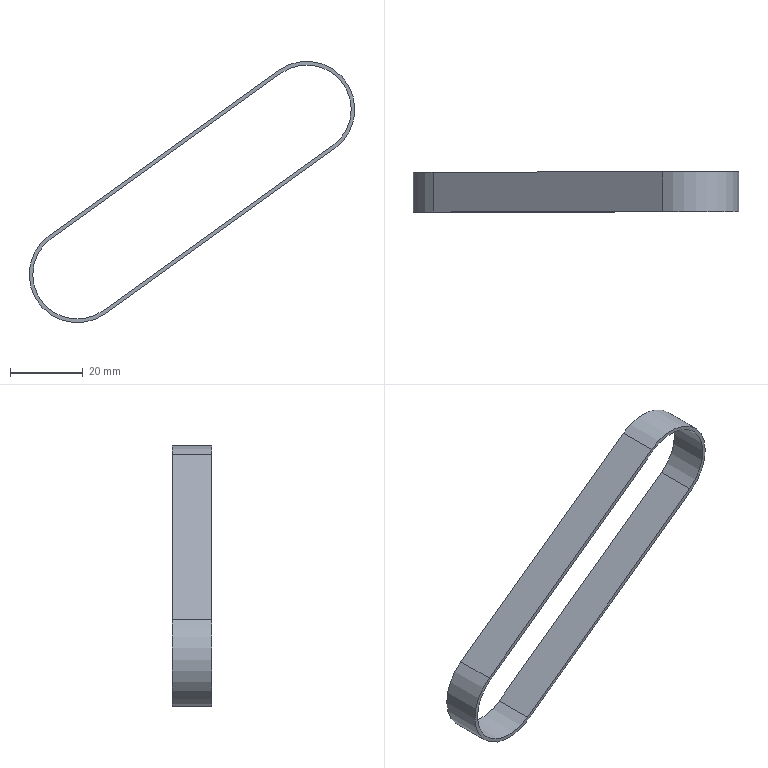Component | NX | BELT | 1 solid | 10 faces | box 89.82 x 11 x 72.05 mm | volume 2597 mm3 | plane 6 | cylinder 4 | commonest cylinder face diameters 26.5 x2 24.5 x2
STEP:
#1=CARTESIAN_POINT('',(0.,0.,0.));
#2=DIRECTION('',(0.,0.,1.));
#3=DIRECTION('',(1.,0.,0.));
#4=AXIS2_PLACEMENT_3D('',#1,#2,#3);
#5=CARTESIAN_POINT('',(-439.414,-35.6,389.312));
#6=VERTEX_POINT('',#5);
#7=CARTESIAN_POINT('',(-376.097,-35.6,434.863));
#8=VERTEX_POINT('',#7);
#9=CARTESIAN_POINT('',(-439.414,-35.6,389.312));
#10=DIRECTION('',(0.8118,0.,0.584));
#11=VECTOR('',#10,1.);
#12=LINE('',#9,#11);
#13=CARTESIAN_POINT('',(-438.83,-35.6,388.5));
#14=DIRECTION('',(0.,-1.,0.));
#15=DIRECTION('',(0.8118,0.,0.584));
#16=AXIS2_PLACEMENT_3D('',#13,#14,#15);
#17=PLANE('',#16);
#18=CARTESIAN_POINT('',(-0.,1.));
#19=DIRECTION('',(1.,0.));
#20=VECTOR('',#19,1.);
#21=LINE('',#18,#20);
#22=(GEOMETRIC_REPRESENTATION_CONTEXT(2)PARAMETRIC_REPRESENTATION_CONTEXT()REPRESENTATION_CONTEXT('',''));
#23=DEFINITIONAL_REPRESENTATION('',(#21),#22);
#24=PCURVE('',#17,#23);
#25=CARTESIAN_POINT('',(-439.414,-46.6,389.312));
#26=DIRECTION('',(-0.584,0.,0.8118));
#27=DIRECTION('',(0.,1.,0.));
#28=AXIS2_PLACEMENT_3D('',#25,#26,#27);
#29=PLANE('',#28);
#30=CARTESIAN_POINT('',(11.,0.));
#31=DIRECTION('',(0.,-1.));
#32=VECTOR('',#31,1.);
#33=LINE('',#30,#32);
#34=(GEOMETRIC_REPRESENTATION_CONTEXT(2)PARAMETRIC_REPRESENTATION_CONTEXT()REPRESENTATION_CONTEXT('',''));
#35=DEFINITIONAL_REPRESENTATION('',(#33),#34);
#36=PCURVE('',#29,#35);
#37=SURFACE_CURVE('',#12,(#24,#36),.PCURVE_S1.);
#38=EDGE_CURVE('',#6,#8,#37,.T.);
#39=ORIENTED_EDGE('',*,*,#38,.T.);
#40=CARTESIAN_POINT('',(-360.621,-35.6,413.352));
#41=VERTEX_POINT('',#40);
#42=CARTESIAN_POINT('',(-368.359,-35.6,424.108));
#43=DIRECTION('',(0.,1.,0.));
#44=DIRECTION('',(-0.8118,0.,-0.584));
#45=AXIS2_PLACEMENT_3D('',#42,#43,#44);
#46=CIRCLE('',#45,13.25);
#47=CARTESIAN_POINT('',(64.75,-12.25));
#48=CARTESIAN_POINT('',(64.75,10.7));
#49=CARTESIAN_POINT('',(84.625,-0.7752));
#50=CARTESIAN_POINT('',(104.5,-12.25));
#51=CARTESIAN_POINT('',(84.625,-23.725));
#52=CARTESIAN_POINT('',(64.75,-35.2));
#53=CARTESIAN_POINT('',(64.75,-12.25));
#54=(BOUNDED_CURVE()B_SPLINE_CURVE(2,(#47,#48,#49,#50,#51,#52,#53),.UNSPECIFIED.,.T.,.F.)B_SPLINE_CURVE_WITH_KNOTS((1,2,2,2,2,1),(-2.094,0.,2.094,4.189,6.283,8.378),.UNSPECIFIED.)CURVE()GEOMETRIC_REPRESENTATION_ITEM()RATIONAL_B_SPLINE_CURVE((1.,0.5,1.,0.5,1.,0.5,1.))REPRESENTATION_ITEM(''));
#55=(GEOMETRIC_REPRESENTATION_CONTEXT(2)PARAMETRIC_REPRESENTATION_CONTEXT()REPRESENTATION_CONTEXT('',''));
#56=DEFINITIONAL_REPRESENTATION('',(#54),#55);
#57=PCURVE('',#17,#56);
#58=CARTESIAN_POINT('',(-368.359,-46.6,424.108));
#59=DIRECTION('',(0.,1.,0.));
#60=DIRECTION('',(-0.8118,0.,-0.584));
#61=AXIS2_PLACEMENT_3D('',#58,#59,#60);
#62=CYLINDRICAL_SURFACE('',#61,13.25);
#63=CARTESIAN_POINT('',(0.,11.));
#64=DIRECTION('',(1.,0.));
#65=VECTOR('',#64,1.);
#66=LINE('',#63,#65);
#67=(GEOMETRIC_REPRESENTATION_CONTEXT(2)PARAMETRIC_REPRESENTATION_CONTEXT()REPRESENTATION_CONTEXT('',''));
#68=DEFINITIONAL_REPRESENTATION('',(#66),#67);
#69=PCURVE('',#62,#68);
#70=SURFACE_CURVE('',#46,(#57,#69),.PCURVE_S1.);
#71=EDGE_CURVE('',#8,#41,#70,.T.);
#72=ORIENTED_EDGE('',*,*,#71,.T.);
#73=CARTESIAN_POINT('',(-423.938,-35.6,367.8));
#74=VERTEX_POINT('',#73);
#75=CARTESIAN_POINT('',(-360.621,-35.6,413.352));
#76=DIRECTION('',(-0.8118,0.,-0.584));
#77=VECTOR('',#76,1.);
#78=LINE('',#75,#77);
#79=CARTESIAN_POINT('',(78.,-25.5));
#80=DIRECTION('',(-1.,0.));
#81=VECTOR('',#80,1.);
#82=LINE('',#79,#81);
#83=(GEOMETRIC_REPRESENTATION_CONTEXT(2)PARAMETRIC_REPRESENTATION_CONTEXT()REPRESENTATION_CONTEXT('',''));
#84=DEFINITIONAL_REPRESENTATION('',(#82),#83);
#85=PCURVE('',#17,#84);
#86=CARTESIAN_POINT('',(-360.621,-46.6,413.352));
#87=DIRECTION('',(0.584,0.,-0.8118));
#88=DIRECTION('',(0.,-1.,0.));
#89=AXIS2_PLACEMENT_3D('',#86,#87,#88);
#90=PLANE('',#89);
#91=CARTESIAN_POINT('',(-11.,0.));
#92=DIRECTION('',(0.,1.));
#93=VECTOR('',#92,1.);
#94=LINE('',#91,#93);
#95=(GEOMETRIC_REPRESENTATION_CONTEXT(2)PARAMETRIC_REPRESENTATION_CONTEXT()REPRESENTATION_CONTEXT('',''));
#96=DEFINITIONAL_REPRESENTATION('',(#94),#95);
#97=PCURVE('',#90,#96);
#98=SURFACE_CURVE('',#78,(#85,#97),.PCURVE_S1.);
#99=EDGE_CURVE('',#41,#74,#98,.T.);
#100=ORIENTED_EDGE('',*,*,#99,.T.);
#101=CARTESIAN_POINT('',(-431.676,-35.6,378.556));
#102=DIRECTION('',(0.,1.,0.));
#103=DIRECTION('',(-0.8118,0.,-0.584));
#104=AXIS2_PLACEMENT_3D('',#101,#102,#103);
#105=CIRCLE('',#104,13.25);
#106=CARTESIAN_POINT('',(-13.25,-12.25));
#107=CARTESIAN_POINT('',(-13.25,10.7));
#108=CARTESIAN_POINT('',(6.625,-0.7752));
#109=CARTESIAN_POINT('',(26.5,-12.25));
#110=CARTESIAN_POINT('',(6.625,-23.725));
#111=CARTESIAN_POINT('',(-13.25,-35.2));
#112=CARTESIAN_POINT('',(-13.25,-12.25));
#113=(BOUNDED_CURVE()B_SPLINE_CURVE(2,(#106,#107,#108,#109,#110,#111,#112),.UNSPECIFIED.,.T.,.F.)B_SPLINE_CURVE_WITH_KNOTS((1,2,2,2,2,1),(-2.094,0.,2.094,4.189,6.283,8.378),.UNSPECIFIED.)CURVE()GEOMETRIC_REPRESENTATION_ITEM()RATIONAL_B_SPLINE_CURVE((1.,0.5,1.,0.5,1.,0.5,1.))REPRESENTATION_ITEM(''));
#114=(GEOMETRIC_REPRESENTATION_CONTEXT(2)PARAMETRIC_REPRESENTATION_CONTEXT()REPRESENTATION_CONTEXT('',''));
#115=DEFINITIONAL_REPRESENTATION('',(#113),#114);
#116=PCURVE('',#17,#115);
#117=CARTESIAN_POINT('',(-431.676,-46.6,378.556));
#118=DIRECTION('',(0.,1.,0.));
#119=DIRECTION('',(-0.8118,0.,-0.584));
#120=AXIS2_PLACEMENT_3D('',#117,#118,#119);
#121=CYLINDRICAL_SURFACE('',#120,13.25);
#122=CARTESIAN_POINT('',(0.,11.));
#123=DIRECTION('',(1.,0.));
#124=VECTOR('',#123,1.);
#125=LINE('',#122,#124);
#126=(GEOMETRIC_REPRESENTATION_CONTEXT(2)PARAMETRIC_REPRESENTATION_CONTEXT()REPRESENTATION_CONTEXT('',''));
#127=DEFINITIONAL_REPRESENTATION('',(#125),#126);
#128=PCURVE('',#121,#127);
#129=SURFACE_CURVE('',#105,(#116,#128),.PCURVE_S1.);
#130=EDGE_CURVE('',#74,#6,#129,.T.);
#131=ORIENTED_EDGE('',*,*,#130,.T.);
#132=EDGE_LOOP('',(#39,#72,#100,#131));
#133=FACE_BOUND('',#132,.T.);
#134=CARTESIAN_POINT('',(-438.83,-35.6,388.5));
#135=VERTEX_POINT('',#134);
#136=CARTESIAN_POINT('',(-375.513,-35.6,434.052));
#137=VERTEX_POINT('',#136);
#138=CARTESIAN_POINT('',(-438.83,-35.6,388.5));
#139=DIRECTION('',(0.8118,0.,0.584));
#140=VECTOR('',#139,1.);
#141=LINE('',#138,#140);
#142=CARTESIAN_POINT('',(0.,0.));
#143=DIRECTION('',(1.,0.));
#144=VECTOR('',#143,1.);
#145=LINE('',#142,#144);
#146=(GEOMETRIC_REPRESENTATION_CONTEXT(2)PARAMETRIC_REPRESENTATION_CONTEXT()REPRESENTATION_CONTEXT('',''));
#147=DEFINITIONAL_REPRESENTATION('',(#145),#146);
#148=PCURVE('',#17,#147);
#149=CARTESIAN_POINT('',(-438.83,-46.6,388.5));
#150=DIRECTION('',(-0.584,0.,0.8118));
#151=DIRECTION('',(0.,1.,0.));
#152=AXIS2_PLACEMENT_3D('',#149,#150,#151);
#153=PLANE('',#152);
#154=CARTESIAN_POINT('',(11.,0.));
#155=DIRECTION('',(0.,-1.));
#156=VECTOR('',#155,1.);
#157=LINE('',#154,#156);
#158=(GEOMETRIC_REPRESENTATION_CONTEXT(2)PARAMETRIC_REPRESENTATION_CONTEXT()REPRESENTATION_CONTEXT('',''));
#159=DEFINITIONAL_REPRESENTATION('',(#157),#158);
#160=PCURVE('',#153,#159);
#161=SURFACE_CURVE('',#141,(#148,#160),.PCURVE_S1.);
#162=EDGE_CURVE('',#135,#137,#161,.T.);
#163=ORIENTED_EDGE('',*,*,#162,.F.);
#164=CARTESIAN_POINT('',(-424.522,-35.6,368.612));
#165=VERTEX_POINT('',#164);
#166=CARTESIAN_POINT('',(-431.676,-35.6,378.556));
#167=DIRECTION('',(0.,1.,0.));
#168=DIRECTION('',(-0.8118,0.,-0.584));
#169=AXIS2_PLACEMENT_3D('',#166,#167,#168);
#170=CIRCLE('',#169,12.25);
#171=CARTESIAN_POINT('',(-12.25,-12.25));
#172=CARTESIAN_POINT('',(-12.25,8.968));
#173=CARTESIAN_POINT('',(6.125,-1.641));
#174=CARTESIAN_POINT('',(24.5,-12.25));
#175=CARTESIAN_POINT('',(6.125,-22.859));
#176=CARTESIAN_POINT('',(-12.25,-33.468));
#177=CARTESIAN_POINT('',(-12.25,-12.25));
#178=(BOUNDED_CURVE()B_SPLINE_CURVE(2,(#171,#172,#173,#174,#175,#176,#177),.UNSPECIFIED.,.T.,.F.)B_SPLINE_CURVE_WITH_KNOTS((1,2,2,2,2,1),(-2.094,0.,2.094,4.189,6.283,8.378),.UNSPECIFIED.)CURVE()GEOMETRIC_REPRESENTATION_ITEM()RATIONAL_B_SPLINE_CURVE((1.,0.5,1.,0.5,1.,0.5,1.))REPRESENTATION_ITEM(''));
#179=(GEOMETRIC_REPRESENTATION_CONTEXT(2)PARAMETRIC_REPRESENTATION_CONTEXT()REPRESENTATION_CONTEXT('',''));
#180=DEFINITIONAL_REPRESENTATION('',(#178),#179);
#181=PCURVE('',#17,#180);
#182=CARTESIAN_POINT('',(-431.676,-46.6,378.556));
#183=DIRECTION('',(0.,1.,0.));
#184=DIRECTION('',(-0.8118,0.,-0.584));
#185=AXIS2_PLACEMENT_3D('',#182,#183,#184);
#186=CYLINDRICAL_SURFACE('',#185,12.25);
#187=CARTESIAN_POINT('',(-6.283,11.));
#188=DIRECTION('',(1.,0.));
#189=VECTOR('',#188,1.);
#190=LINE('',#187,#189);
#191=(GEOMETRIC_REPRESENTATION_CONTEXT(2)PARAMETRIC_REPRESENTATION_CONTEXT()REPRESENTATION_CONTEXT('',''));
#192=DEFINITIONAL_REPRESENTATION('',(#190),#191);
#193=PCURVE('',#186,#192);
#194=SURFACE_CURVE('',#170,(#181,#193),.PCURVE_S1.);
#195=EDGE_CURVE('',#165,#135,#194,.T.);
#196=ORIENTED_EDGE('',*,*,#195,.F.);
#197=CARTESIAN_POINT('',(-361.205,-35.6,414.164));
#198=VERTEX_POINT('',#197);
#199=CARTESIAN_POINT('',(-361.205,-35.6,414.164));
#200=DIRECTION('',(-0.8118,0.,-0.584));
#201=VECTOR('',#200,1.);
#202=LINE('',#199,#201);
#203=CARTESIAN_POINT('',(78.,-24.5));
#204=DIRECTION('',(-1.,0.));
#205=VECTOR('',#204,1.);
#206=LINE('',#203,#205);
#207=(GEOMETRIC_REPRESENTATION_CONTEXT(2)PARAMETRIC_REPRESENTATION_CONTEXT()REPRESENTATION_CONTEXT('',''));
#208=DEFINITIONAL_REPRESENTATION('',(#206),#207);
#209=PCURVE('',#17,#208);
#210=CARTESIAN_POINT('',(-361.205,-46.6,414.164));
#211=DIRECTION('',(0.584,0.,-0.8118));
#212=DIRECTION('',(0.,-1.,0.));
#213=AXIS2_PLACEMENT_3D('',#210,#211,#212);
#214=PLANE('',#213);
#215=CARTESIAN_POINT('',(-11.,0.));
#216=DIRECTION('',(0.,1.));
#217=VECTOR('',#216,1.);
#218=LINE('',#215,#217);
#219=(GEOMETRIC_REPRESENTATION_CONTEXT(2)PARAMETRIC_REPRESENTATION_CONTEXT()REPRESENTATION_CONTEXT('',''));
#220=DEFINITIONAL_REPRESENTATION('',(#218),#219);
#221=PCURVE('',#214,#220);
#222=SURFACE_CURVE('',#202,(#209,#221),.PCURVE_S1.);
#223=EDGE_CURVE('',#198,#165,#222,.T.);
#224=ORIENTED_EDGE('',*,*,#223,.F.);
#225=CARTESIAN_POINT('',(-368.359,-35.6,424.108));
#226=DIRECTION('',(0.,1.,0.));
#227=DIRECTION('',(-0.8118,0.,-0.584));
#228=AXIS2_PLACEMENT_3D('',#225,#226,#227);
#229=CIRCLE('',#228,12.25);
#230=CARTESIAN_POINT('',(65.75,-12.25));
#231=CARTESIAN_POINT('',(65.75,8.968));
#232=CARTESIAN_POINT('',(84.125,-1.641));
#233=CARTESIAN_POINT('',(102.5,-12.25));
#234=CARTESIAN_POINT('',(84.125,-22.859));
#235=CARTESIAN_POINT('',(65.75,-33.468));
#236=CARTESIAN_POINT('',(65.75,-12.25));
#237=(BOUNDED_CURVE()B_SPLINE_CURVE(2,(#230,#231,#232,#233,#234,#235,#236),.UNSPECIFIED.,.T.,.F.)B_SPLINE_CURVE_WITH_KNOTS((1,2,2,2,2,1),(-2.094,0.,2.094,4.189,6.283,8.378),.UNSPECIFIED.)CURVE()GEOMETRIC_REPRESENTATION_ITEM()RATIONAL_B_SPLINE_CURVE((1.,0.5,1.,0.5,1.,0.5,1.))REPRESENTATION_ITEM(''));
#238=(GEOMETRIC_REPRESENTATION_CONTEXT(2)PARAMETRIC_REPRESENTATION_CONTEXT()REPRESENTATION_CONTEXT('',''));
#239=DEFINITIONAL_REPRESENTATION('',(#237),#238);
#240=PCURVE('',#17,#239);
#241=CARTESIAN_POINT('',(-368.359,-46.6,424.108));
#242=DIRECTION('',(0.,1.,0.));
#243=DIRECTION('',(-0.8118,0.,-0.584));
#244=AXIS2_PLACEMENT_3D('',#241,#242,#243);
#245=CYLINDRICAL_SURFACE('',#244,12.25);
#246=CARTESIAN_POINT('',(-0.,11.));
#247=DIRECTION('',(1.,0.));
#248=VECTOR('',#247,1.);
#249=LINE('',#246,#248);
#250=(GEOMETRIC_REPRESENTATION_CONTEXT(2)PARAMETRIC_REPRESENTATION_CONTEXT()REPRESENTATION_CONTEXT('',''));
#251=DEFINITIONAL_REPRESENTATION('',(#249),#250);
#252=PCURVE('',#245,#251);
#253=SURFACE_CURVE('',#229,(#240,#252),.PCURVE_S1.);
#254=EDGE_CURVE('',#137,#198,#253,.T.);
#255=ORIENTED_EDGE('',*,*,#254,.F.);
#256=EDGE_LOOP('',(#163,#196,#224,#255));
#257=FACE_BOUND('',#256,.T.);
#258=ADVANCED_FACE('',(#133,#257),#17,.F.);
#259=CARTESIAN_POINT('',(-360.621,-46.6,413.352));
#260=VERTEX_POINT('',#259);
#261=CARTESIAN_POINT('',(-423.938,-46.6,367.8));
#262=VERTEX_POINT('',#261);
#263=CARTESIAN_POINT('',(-360.621,-46.6,413.352));
#264=DIRECTION('',(-0.8118,0.,-0.584));
#265=VECTOR('',#264,1.);
#266=LINE('',#263,#265);
#267=CARTESIAN_POINT('',(-361.205,-46.6,414.164));
#268=DIRECTION('',(0.,-1.,0.));
#269=DIRECTION('',(-0.8118,0.,-0.584));
#270=AXIS2_PLACEMENT_3D('',#267,#268,#269);
#271=PLANE('',#270);
#272=CARTESIAN_POINT('',(0.,1.));
#273=DIRECTION('',(1.,0.));
#274=VECTOR('',#273,1.);
#275=LINE('',#272,#274);
#276=(GEOMETRIC_REPRESENTATION_CONTEXT(2)PARAMETRIC_REPRESENTATION_CONTEXT()REPRESENTATION_CONTEXT('',''));
#277=DEFINITIONAL_REPRESENTATION('',(#275),#276);
#278=PCURVE('',#271,#277);
#279=CARTESIAN_POINT('',(0.,0.));
#280=DIRECTION('',(0.,1.));
#281=VECTOR('',#280,1.);
#282=LINE('',#279,#281);
#283=(GEOMETRIC_REPRESENTATION_CONTEXT(2)PARAMETRIC_REPRESENTATION_CONTEXT()REPRESENTATION_CONTEXT('',''));
#284=DEFINITIONAL_REPRESENTATION('',(#282),#283);
#285=PCURVE('',#90,#284);
#286=SURFACE_CURVE('',#266,(#278,#285),.PCURVE_S1.);
#287=EDGE_CURVE('',#260,#262,#286,.T.);
#288=ORIENTED_EDGE('',*,*,#287,.F.);
#289=CARTESIAN_POINT('',(-376.097,-46.6,434.863));
#290=VERTEX_POINT('',#289);
#291=CARTESIAN_POINT('',(-368.359,-46.6,424.108));
#292=DIRECTION('',(0.,1.,0.));
#293=DIRECTION('',(-0.8118,0.,-0.584));
#294=AXIS2_PLACEMENT_3D('',#291,#292,#293);
#295=CIRCLE('',#294,13.25);
#296=CARTESIAN_POINT('',(13.25,-12.25));
#297=CARTESIAN_POINT('',(13.25,-35.2));
#298=CARTESIAN_POINT('',(-6.625,-23.725));
#299=CARTESIAN_POINT('',(-26.5,-12.25));
#300=CARTESIAN_POINT('',(-6.625,-0.7752));
#301=CARTESIAN_POINT('',(13.25,10.7));
#302=CARTESIAN_POINT('',(13.25,-12.25));
#303=(BOUNDED_CURVE()B_SPLINE_CURVE(2,(#296,#297,#298,#299,#300,#301,#302),.UNSPECIFIED.,.T.,.F.)B_SPLINE_CURVE_WITH_KNOTS((1,2,2,2,2,1),(-2.094,0.,2.094,4.189,6.283,8.378),.UNSPECIFIED.)CURVE()GEOMETRIC_REPRESENTATION_ITEM()RATIONAL_B_SPLINE_CURVE((1.,0.5,1.,0.5,1.,0.5,1.))REPRESENTATION_ITEM(''));
#304=(GEOMETRIC_REPRESENTATION_CONTEXT(2)PARAMETRIC_REPRESENTATION_CONTEXT()REPRESENTATION_CONTEXT('',''));
#305=DEFINITIONAL_REPRESENTATION('',(#303),#304);
#306=PCURVE('',#271,#305);
#307=CARTESIAN_POINT('',(0.,0.));
#308=DIRECTION('',(1.,0.));
#309=VECTOR('',#308,1.);
#310=LINE('',#307,#309);
#311=(GEOMETRIC_REPRESENTATION_CONTEXT(2)PARAMETRIC_REPRESENTATION_CONTEXT()REPRESENTATION_CONTEXT('',''));
#312=DEFINITIONAL_REPRESENTATION('',(#310),#311);
#313=PCURVE('',#62,#312);
#314=SURFACE_CURVE('',#295,(#306,#313),.PCURVE_S1.);
#315=EDGE_CURVE('',#290,#260,#314,.T.);
#316=ORIENTED_EDGE('',*,*,#315,.F.);
#317=CARTESIAN_POINT('',(-439.414,-46.6,389.312));
#318=VERTEX_POINT('',#317);
#319=CARTESIAN_POINT('',(-439.414,-46.6,389.312));
#320=DIRECTION('',(0.8118,0.,0.584));
#321=VECTOR('',#320,1.);
#322=LINE('',#319,#321);
#323=CARTESIAN_POINT('',(78.,-25.5));
#324=DIRECTION('',(-1.,0.));
#325=VECTOR('',#324,1.);
#326=LINE('',#323,#325);
#327=(GEOMETRIC_REPRESENTATION_CONTEXT(2)PARAMETRIC_REPRESENTATION_CONTEXT()REPRESENTATION_CONTEXT('',''));
#328=DEFINITIONAL_REPRESENTATION('',(#326),#327);
#329=PCURVE('',#271,#328);
#330=CARTESIAN_POINT('',(0.,0.));
#331=DIRECTION('',(0.,-1.));
#332=VECTOR('',#331,1.);
#333=LINE('',#330,#332);
#334=(GEOMETRIC_REPRESENTATION_CONTEXT(2)PARAMETRIC_REPRESENTATION_CONTEXT()REPRESENTATION_CONTEXT('',''));
#335=DEFINITIONAL_REPRESENTATION('',(#333),#334);
#336=PCURVE('',#29,#335);
#337=SURFACE_CURVE('',#322,(#329,#336),.PCURVE_S1.);
#338=EDGE_CURVE('',#318,#290,#337,.T.);
#339=ORIENTED_EDGE('',*,*,#338,.F.);
#340=CARTESIAN_POINT('',(-431.676,-46.6,378.556));
#341=DIRECTION('',(0.,1.,0.));
#342=DIRECTION('',(-0.8118,0.,-0.584));
#343=AXIS2_PLACEMENT_3D('',#340,#341,#342);
#344=CIRCLE('',#343,13.25);
#345=CARTESIAN_POINT('',(91.25,-12.25));
#346=CARTESIAN_POINT('',(91.25,-35.2));
#347=CARTESIAN_POINT('',(71.375,-23.725));
#348=CARTESIAN_POINT('',(51.5,-12.25));
#349=CARTESIAN_POINT('',(71.375,-0.7752));
#350=CARTESIAN_POINT('',(91.25,10.7));
#351=CARTESIAN_POINT('',(91.25,-12.25));
#352=(BOUNDED_CURVE()B_SPLINE_CURVE(2,(#345,#346,#347,#348,#349,#350,#351),.UNSPECIFIED.,.T.,.F.)B_SPLINE_CURVE_WITH_KNOTS((1,2,2,2,2,1),(-2.094,0.,2.094,4.189,6.283,8.378),.UNSPECIFIED.)CURVE()GEOMETRIC_REPRESENTATION_ITEM()RATIONAL_B_SPLINE_CURVE((1.,0.5,1.,0.5,1.,0.5,1.))REPRESENTATION_ITEM(''));
#353=(GEOMETRIC_REPRESENTATION_CONTEXT(2)PARAMETRIC_REPRESENTATION_CONTEXT()REPRESENTATION_CONTEXT('',''));
#354=DEFINITIONAL_REPRESENTATION('',(#352),#353);
#355=PCURVE('',#271,#354);
#356=CARTESIAN_POINT('',(0.,0.));
#357=DIRECTION('',(1.,0.));
#358=VECTOR('',#357,1.);
#359=LINE('',#356,#358);
#360=(GEOMETRIC_REPRESENTATION_CONTEXT(2)PARAMETRIC_REPRESENTATION_CONTEXT()REPRESENTATION_CONTEXT('',''));
#361=DEFINITIONAL_REPRESENTATION('',(#359),#360);
#362=PCURVE('',#121,#361);
#363=SURFACE_CURVE('',#344,(#355,#362),.PCURVE_S1.);
#364=EDGE_CURVE('',#262,#318,#363,.T.);
#365=ORIENTED_EDGE('',*,*,#364,.F.);
#366=EDGE_LOOP('',(#288,#316,#339,#365));
#367=FACE_BOUND('',#366,.T.);
#368=CARTESIAN_POINT('',(-361.205,-46.6,414.164));
#369=VERTEX_POINT('',#368);
#370=CARTESIAN_POINT('',(-424.522,-46.6,368.612));
#371=VERTEX_POINT('',#370);
#372=CARTESIAN_POINT('',(-361.205,-46.6,414.164));
#373=DIRECTION('',(-0.8118,0.,-0.584));
#374=VECTOR('',#373,1.);
#375=LINE('',#372,#374);
#376=CARTESIAN_POINT('',(0.,0.));
#377=DIRECTION('',(1.,0.));
#378=VECTOR('',#377,1.);
#379=LINE('',#376,#378);
#380=(GEOMETRIC_REPRESENTATION_CONTEXT(2)PARAMETRIC_REPRESENTATION_CONTEXT()REPRESENTATION_CONTEXT('',''));
#381=DEFINITIONAL_REPRESENTATION('',(#379),#380);
#382=PCURVE('',#271,#381);
#383=CARTESIAN_POINT('',(0.,0.));
#384=DIRECTION('',(0.,1.));
#385=VECTOR('',#384,1.);
#386=LINE('',#383,#385);
#387=(GEOMETRIC_REPRESENTATION_CONTEXT(2)PARAMETRIC_REPRESENTATION_CONTEXT()REPRESENTATION_CONTEXT('',''));
#388=DEFINITIONAL_REPRESENTATION('',(#386),#387);
#389=PCURVE('',#214,#388);
#390=SURFACE_CURVE('',#375,(#382,#389),.PCURVE_S1.);
#391=EDGE_CURVE('',#369,#371,#390,.T.);
#392=ORIENTED_EDGE('',*,*,#391,.T.);
#393=CARTESIAN_POINT('',(-438.83,-46.6,388.5));
#394=VERTEX_POINT('',#393);
#395=CARTESIAN_POINT('',(-431.676,-46.6,378.556));
#396=DIRECTION('',(0.,1.,0.));
#397=DIRECTION('',(-0.8118,0.,-0.584));
#398=AXIS2_PLACEMENT_3D('',#395,#396,#397);
#399=CIRCLE('',#398,12.25);
#400=CARTESIAN_POINT('',(90.25,-12.25));
#401=CARTESIAN_POINT('',(90.25,-33.468));
#402=CARTESIAN_POINT('',(71.875,-22.859));
#403=CARTESIAN_POINT('',(53.5,-12.25));
#404=CARTESIAN_POINT('',(71.875,-1.641));
#405=CARTESIAN_POINT('',(90.25,8.968));
#406=CARTESIAN_POINT('',(90.25,-12.25));
#407=(BOUNDED_CURVE()B_SPLINE_CURVE(2,(#400,#401,#402,#403,#404,#405,#406),.UNSPECIFIED.,.T.,.F.)B_SPLINE_CURVE_WITH_KNOTS((1,2,2,2,2,1),(-2.094,0.,2.094,4.189,6.283,8.378),.UNSPECIFIED.)CURVE()GEOMETRIC_REPRESENTATION_ITEM()RATIONAL_B_SPLINE_CURVE((1.,0.5,1.,0.5,1.,0.5,1.))REPRESENTATION_ITEM(''));
#408=(GEOMETRIC_REPRESENTATION_CONTEXT(2)PARAMETRIC_REPRESENTATION_CONTEXT()REPRESENTATION_CONTEXT('',''));
#409=DEFINITIONAL_REPRESENTATION('',(#407),#408);
#410=PCURVE('',#271,#409);
#411=CARTESIAN_POINT('',(-6.283,0.));
#412=DIRECTION('',(1.,0.));
#413=VECTOR('',#412,1.);
#414=LINE('',#411,#413);
#415=(GEOMETRIC_REPRESENTATION_CONTEXT(2)PARAMETRIC_REPRESENTATION_CONTEXT()REPRESENTATION_CONTEXT('',''));
#416=DEFINITIONAL_REPRESENTATION('',(#414),#415);
#417=PCURVE('',#186,#416);
#418=SURFACE_CURVE('',#399,(#410,#417),.PCURVE_S1.);
#419=EDGE_CURVE('',#371,#394,#418,.T.);
#420=ORIENTED_EDGE('',*,*,#419,.T.);
#421=CARTESIAN_POINT('',(-375.513,-46.6,434.052));
#422=VERTEX_POINT('',#421);
#423=CARTESIAN_POINT('',(-438.83,-46.6,388.5));
#424=DIRECTION('',(0.8118,0.,0.584));
#425=VECTOR('',#424,1.);
#426=LINE('',#423,#425);
#427=CARTESIAN_POINT('',(78.,-24.5));
#428=DIRECTION('',(-1.,0.));
#429=VECTOR('',#428,1.);
#430=LINE('',#427,#429);
#431=(GEOMETRIC_REPRESENTATION_CONTEXT(2)PARAMETRIC_REPRESENTATION_CONTEXT()REPRESENTATION_CONTEXT('',''));
#432=DEFINITIONAL_REPRESENTATION('',(#430),#431);
#433=PCURVE('',#271,#432);
#434=CARTESIAN_POINT('',(0.,0.));
#435=DIRECTION('',(0.,-1.));
#436=VECTOR('',#435,1.);
#437=LINE('',#434,#436);
#438=(GEOMETRIC_REPRESENTATION_CONTEXT(2)PARAMETRIC_REPRESENTATION_CONTEXT()REPRESENTATION_CONTEXT('',''));
#439=DEFINITIONAL_REPRESENTATION('',(#437),#438);
#440=PCURVE('',#153,#439);
#441=SURFACE_CURVE('',#426,(#433,#440),.PCURVE_S1.);
#442=EDGE_CURVE('',#394,#422,#441,.T.);
#443=ORIENTED_EDGE('',*,*,#442,.T.);
#444=CARTESIAN_POINT('',(-368.359,-46.6,424.108));
#445=DIRECTION('',(0.,1.,0.));
#446=DIRECTION('',(-0.8118,0.,-0.584));
#447=AXIS2_PLACEMENT_3D('',#444,#445,#446);
#448=CIRCLE('',#447,12.25);
#449=CARTESIAN_POINT('',(12.25,-12.25));
#450=CARTESIAN_POINT('',(12.25,-33.468));
#451=CARTESIAN_POINT('',(-6.125,-22.859));
#452=CARTESIAN_POINT('',(-24.5,-12.25));
#453=CARTESIAN_POINT('',(-6.125,-1.641));
#454=CARTESIAN_POINT('',(12.25,8.968));
#455=CARTESIAN_POINT('',(12.25,-12.25));
#456=(BOUNDED_CURVE()B_SPLINE_CURVE(2,(#449,#450,#451,#452,#453,#454,#455),.UNSPECIFIED.,.T.,.F.)B_SPLINE_CURVE_WITH_KNOTS((1,2,2,2,2,1),(-2.094,0.,2.094,4.189,6.283,8.378),.UNSPECIFIED.)CURVE()GEOMETRIC_REPRESENTATION_ITEM()RATIONAL_B_SPLINE_CURVE((1.,0.5,1.,0.5,1.,0.5,1.))REPRESENTATION_ITEM(''));
#457=(GEOMETRIC_REPRESENTATION_CONTEXT(2)PARAMETRIC_REPRESENTATION_CONTEXT()REPRESENTATION_CONTEXT('',''));
#458=DEFINITIONAL_REPRESENTATION('',(#456),#457);
#459=PCURVE('',#271,#458);
#460=CARTESIAN_POINT('',(-0.,0.));
#461=DIRECTION('',(1.,0.));
#462=VECTOR('',#461,1.);
#463=LINE('',#460,#462);
#464=(GEOMETRIC_REPRESENTATION_CONTEXT(2)PARAMETRIC_REPRESENTATION_CONTEXT()REPRESENTATION_CONTEXT('',''));
#465=DEFINITIONAL_REPRESENTATION('',(#463),#464);
#466=PCURVE('',#245,#465);
#467=SURFACE_CURVE('',#448,(#459,#466),.PCURVE_S1.);
#468=EDGE_CURVE('',#422,#369,#467,.T.);
#469=ORIENTED_EDGE('',*,*,#468,.T.);
#470=EDGE_LOOP('',(#392,#420,#443,#469));
#471=FACE_BOUND('',#470,.T.);
#472=ADVANCED_FACE('',(#367,#471),#271,.T.);
#473=ORIENTED_EDGE('',*,*,#71,.F.);
#474=CARTESIAN_POINT('',(-376.097,-46.6,434.863));
#475=DIRECTION('',(0.,1.,0.));
#476=VECTOR('',#475,1.);
#477=LINE('',#474,#476);
#478=CARTESIAN_POINT('',(1.571,0.));
#479=DIRECTION('',(0.,1.));
#480=VECTOR('',#479,1.);
#481=LINE('',#478,#480);
#482=(GEOMETRIC_REPRESENTATION_CONTEXT(2)PARAMETRIC_REPRESENTATION_CONTEXT()REPRESENTATION_CONTEXT('',''));
#483=DEFINITIONAL_REPRESENTATION('',(#481),#482);
#484=PCURVE('',#62,#483);
#485=CARTESIAN_POINT('',(0.,-78.));
#486=DIRECTION('',(1.,0.));
#487=VECTOR('',#486,1.);
#488=LINE('',#485,#487);
#489=(GEOMETRIC_REPRESENTATION_CONTEXT(2)PARAMETRIC_REPRESENTATION_CONTEXT()REPRESENTATION_CONTEXT('',''));
#490=DEFINITIONAL_REPRESENTATION('',(#488),#489);
#491=PCURVE('',#29,#490);
#492=SURFACE_CURVE('',#477,(#484,#491),.PCURVE_S1.);
#493=EDGE_CURVE('',#290,#8,#492,.T.);
#494=ORIENTED_EDGE('',*,*,#493,.F.);
#495=ORIENTED_EDGE('',*,*,#315,.T.);
#496=CARTESIAN_POINT('',(-360.621,-46.6,413.352));
#497=DIRECTION('',(0.,1.,0.));
#498=VECTOR('',#497,1.);
#499=LINE('',#496,#498);
#500=CARTESIAN_POINT('',(4.712,0.));
#501=DIRECTION('',(0.,1.));
#502=VECTOR('',#501,1.);
#503=LINE('',#500,#502);
#504=(GEOMETRIC_REPRESENTATION_CONTEXT(2)PARAMETRIC_REPRESENTATION_CONTEXT()REPRESENTATION_CONTEXT('',''));
#505=DEFINITIONAL_REPRESENTATION('',(#503),#504);
#506=PCURVE('',#62,#505);
#507=CARTESIAN_POINT('',(0.,0.));
#508=DIRECTION('',(-1.,0.));
#509=VECTOR('',#508,1.);
#510=LINE('',#507,#509);
#511=(GEOMETRIC_REPRESENTATION_CONTEXT(2)PARAMETRIC_REPRESENTATION_CONTEXT()REPRESENTATION_CONTEXT('',''));
#512=DEFINITIONAL_REPRESENTATION('',(#510),#511);
#513=PCURVE('',#90,#512);
#514=SURFACE_CURVE('',#499,(#506,#513),.PCURVE_S1.);
#515=EDGE_CURVE('',#260,#41,#514,.T.);
#516=ORIENTED_EDGE('',*,*,#515,.T.);
#517=EDGE_LOOP('',(#473,#494,#495,#516));
#518=FACE_BOUND('',#517,.T.);
#519=ADVANCED_FACE('',(#518),#62,.T.);
#520=ORIENTED_EDGE('',*,*,#99,.F.);
#521=ORIENTED_EDGE('',*,*,#515,.F.);
#522=ORIENTED_EDGE('',*,*,#287,.T.);
#523=CARTESIAN_POINT('',(-423.938,-46.6,367.8));
#524=DIRECTION('',(0.,1.,0.));
#525=VECTOR('',#524,1.);
#526=LINE('',#523,#525);
#527=CARTESIAN_POINT('',(0.,78.));
#528=DIRECTION('',(-1.,0.));
#529=VECTOR('',#528,1.);
#530=LINE('',#527,#529);
#531=(GEOMETRIC_REPRESENTATION_CONTEXT(2)PARAMETRIC_REPRESENTATION_CONTEXT()REPRESENTATION_CONTEXT('',''));
#532=DEFINITIONAL_REPRESENTATION('',(#530),#531);
#533=PCURVE('',#90,#532);
#534=CARTESIAN_POINT('',(4.712,0.));
#535=DIRECTION('',(0.,1.));
#536=VECTOR('',#535,1.);
#537=LINE('',#534,#536);
#538=(GEOMETRIC_REPRESENTATION_CONTEXT(2)PARAMETRIC_REPRESENTATION_CONTEXT()REPRESENTATION_CONTEXT('',''));
#539=DEFINITIONAL_REPRESENTATION('',(#537),#538);
#540=PCURVE('',#121,#539);
#541=SURFACE_CURVE('',#526,(#533,#540),.PCURVE_S1.);
#542=EDGE_CURVE('',#262,#74,#541,.T.);
#543=ORIENTED_EDGE('',*,*,#542,.T.);
#544=EDGE_LOOP('',(#520,#521,#522,#543));
#545=FACE_BOUND('',#544,.T.);
#546=ADVANCED_FACE('',(#545),#90,.T.);
#547=ORIENTED_EDGE('',*,*,#130,.F.);
#548=ORIENTED_EDGE('',*,*,#542,.F.);
#549=ORIENTED_EDGE('',*,*,#364,.T.);
#550=CARTESIAN_POINT('',(-439.414,-46.6,389.312));
#551=DIRECTION('',(0.,1.,0.));
#552=VECTOR('',#551,1.);
#553=LINE('',#550,#552);
#554=CARTESIAN_POINT('',(7.854,0.));
#555=DIRECTION('',(0.,1.));
#556=VECTOR('',#555,1.);
#557=LINE('',#554,#556);
#558=(GEOMETRIC_REPRESENTATION_CONTEXT(2)PARAMETRIC_REPRESENTATION_CONTEXT()REPRESENTATION_CONTEXT('',''));
#559=DEFINITIONAL_REPRESENTATION('',(#557),#558);
#560=PCURVE('',#121,#559);
#561=CARTESIAN_POINT('',(0.,0.));
#562=DIRECTION('',(1.,0.));
#563=VECTOR('',#562,1.);
#564=LINE('',#561,#563);
#565=(GEOMETRIC_REPRESENTATION_CONTEXT(2)PARAMETRIC_REPRESENTATION_CONTEXT()REPRESENTATION_CONTEXT('',''));
#566=DEFINITIONAL_REPRESENTATION('',(#564),#565);
#567=PCURVE('',#29,#566);
#568=SURFACE_CURVE('',#553,(#560,#567),.PCURVE_S1.);
#569=EDGE_CURVE('',#318,#6,#568,.T.);
#570=ORIENTED_EDGE('',*,*,#569,.T.);
#571=EDGE_LOOP('',(#547,#548,#549,#570));
#572=FACE_BOUND('',#571,.T.);
#573=ADVANCED_FACE('',(#572),#121,.T.);
#574=ORIENTED_EDGE('',*,*,#38,.F.);
#575=ORIENTED_EDGE('',*,*,#569,.F.);
#576=ORIENTED_EDGE('',*,*,#338,.T.);
#577=ORIENTED_EDGE('',*,*,#493,.T.);
#578=EDGE_LOOP('',(#574,#575,#576,#577));
#579=FACE_BOUND('',#578,.T.);
#580=ADVANCED_FACE('',(#579),#29,.T.);
#581=CARTESIAN_POINT('',(-375.513,-46.6,434.052));
#582=DIRECTION('',(0.,1.,0.));
#583=VECTOR('',#582,1.);
#584=LINE('',#581,#583);
#585=CARTESIAN_POINT('',(1.571,0.));
#586=DIRECTION('',(0.,1.));
#587=VECTOR('',#586,1.);
#588=LINE('',#585,#587);
#589=(GEOMETRIC_REPRESENTATION_CONTEXT(2)PARAMETRIC_REPRESENTATION_CONTEXT()REPRESENTATION_CONTEXT('',''));
#590=DEFINITIONAL_REPRESENTATION('',(#588),#589);
#591=PCURVE('',#245,#590);
#592=CARTESIAN_POINT('',(0.,-78.));
#593=DIRECTION('',(1.,0.));
#594=VECTOR('',#593,1.);
#595=LINE('',#592,#594);
#596=(GEOMETRIC_REPRESENTATION_CONTEXT(2)PARAMETRIC_REPRESENTATION_CONTEXT()REPRESENTATION_CONTEXT('',''));
#597=DEFINITIONAL_REPRESENTATION('',(#595),#596);
#598=PCURVE('',#153,#597);
#599=SURFACE_CURVE('',#584,(#591,#598),.PCURVE_S1.);
#600=EDGE_CURVE('',#422,#137,#599,.T.);
#601=ORIENTED_EDGE('',*,*,#600,.F.);
#602=ORIENTED_EDGE('',*,*,#468,.T.);
#603=CARTESIAN_POINT('',(-361.205,-46.6,414.164));
#604=DIRECTION('',(0.,1.,0.));
#605=VECTOR('',#604,1.);
#606=LINE('',#603,#605);
#607=CARTESIAN_POINT('',(4.712,0.));
#608=DIRECTION('',(0.,1.));
#609=VECTOR('',#608,1.);
#610=LINE('',#607,#609);
#611=(GEOMETRIC_REPRESENTATION_CONTEXT(2)PARAMETRIC_REPRESENTATION_CONTEXT()REPRESENTATION_CONTEXT('',''));
#612=DEFINITIONAL_REPRESENTATION('',(#610),#611);
#613=PCURVE('',#245,#612);
#614=CARTESIAN_POINT('',(0.,0.));
#615=DIRECTION('',(-1.,0.));
#616=VECTOR('',#615,1.);
#617=LINE('',#614,#616);
#618=(GEOMETRIC_REPRESENTATION_CONTEXT(2)PARAMETRIC_REPRESENTATION_CONTEXT()REPRESENTATION_CONTEXT('',''));
#619=DEFINITIONAL_REPRESENTATION('',(#617),#618);
#620=PCURVE('',#214,#619);
#621=SURFACE_CURVE('',#606,(#613,#620),.PCURVE_S1.);
#622=EDGE_CURVE('',#369,#198,#621,.T.);
#623=ORIENTED_EDGE('',*,*,#622,.T.);
#624=ORIENTED_EDGE('',*,*,#254,.F.);
#625=EDGE_LOOP('',(#601,#602,#623,#624));
#626=FACE_BOUND('',#625,.F.);
#627=ADVANCED_FACE('',(#626),#245,.F.);
#628=ORIENTED_EDGE('',*,*,#223,.T.);
#629=CARTESIAN_POINT('',(-424.522,-46.6,368.612));
#630=DIRECTION('',(0.,1.,0.));
#631=VECTOR('',#630,1.);
#632=LINE('',#629,#631);
#633=CARTESIAN_POINT('',(0.,78.));
#634=DIRECTION('',(-1.,0.));
#635=VECTOR('',#634,1.);
#636=LINE('',#633,#635);
#637=(GEOMETRIC_REPRESENTATION_CONTEXT(2)PARAMETRIC_REPRESENTATION_CONTEXT()REPRESENTATION_CONTEXT('',''));
#638=DEFINITIONAL_REPRESENTATION('',(#636),#637);
#639=PCURVE('',#214,#638);
#640=CARTESIAN_POINT('',(-1.571,0.));
#641=DIRECTION('',(0.,1.));
#642=VECTOR('',#641,1.);
#643=LINE('',#640,#642);
#644=(GEOMETRIC_REPRESENTATION_CONTEXT(2)PARAMETRIC_REPRESENTATION_CONTEXT()REPRESENTATION_CONTEXT('',''));
#645=DEFINITIONAL_REPRESENTATION('',(#643),#644);
#646=PCURVE('',#186,#645);
#647=SURFACE_CURVE('',#632,(#639,#646),.PCURVE_S1.);
#648=EDGE_CURVE('',#371,#165,#647,.T.);
#649=ORIENTED_EDGE('',*,*,#648,.F.);
#650=ORIENTED_EDGE('',*,*,#391,.F.);
#651=ORIENTED_EDGE('',*,*,#622,.T.);
#652=EDGE_LOOP('',(#628,#649,#650,#651));
#653=FACE_BOUND('',#652,.T.);
#654=ADVANCED_FACE('',(#653),#214,.F.);
#655=ORIENTED_EDGE('',*,*,#648,.F.);
#656=ORIENTED_EDGE('',*,*,#419,.T.);
#657=CARTESIAN_POINT('',(-438.83,-46.6,388.5));
#658=DIRECTION('',(0.,1.,0.));
#659=VECTOR('',#658,1.);
#660=LINE('',#657,#659);
#661=CARTESIAN_POINT('',(1.571,0.));
#662=DIRECTION('',(0.,1.));
#663=VECTOR('',#662,1.);
#664=LINE('',#661,#663);
#665=(GEOMETRIC_REPRESENTATION_CONTEXT(2)PARAMETRIC_REPRESENTATION_CONTEXT()REPRESENTATION_CONTEXT('',''));
#666=DEFINITIONAL_REPRESENTATION('',(#664),#665);
#667=PCURVE('',#186,#666);
#668=CARTESIAN_POINT('',(0.,0.));
#669=DIRECTION('',(1.,0.));
#670=VECTOR('',#669,1.);
#671=LINE('',#668,#670);
#672=(GEOMETRIC_REPRESENTATION_CONTEXT(2)PARAMETRIC_REPRESENTATION_CONTEXT()REPRESENTATION_CONTEXT('',''));
#673=DEFINITIONAL_REPRESENTATION('',(#671),#672);
#674=PCURVE('',#153,#673);
#675=SURFACE_CURVE('',#660,(#667,#674),.PCURVE_S1.);
#676=EDGE_CURVE('',#394,#135,#675,.T.);
#677=ORIENTED_EDGE('',*,*,#676,.T.);
#678=ORIENTED_EDGE('',*,*,#195,.F.);
#679=EDGE_LOOP('',(#655,#656,#677,#678));
#680=FACE_BOUND('',#679,.F.);
#681=ADVANCED_FACE('',(#680),#186,.F.);
#682=ORIENTED_EDGE('',*,*,#162,.T.);
#683=ORIENTED_EDGE('',*,*,#600,.F.);
#684=ORIENTED_EDGE('',*,*,#442,.F.);
#685=ORIENTED_EDGE('',*,*,#676,.T.);
#686=EDGE_LOOP('',(#682,#683,#684,#685));
#687=FACE_BOUND('',#686,.T.);
#688=ADVANCED_FACE('',(#687),#153,.F.);
#689=CLOSED_SHELL('',(#258,#472,#519,#546,#573,#580,#627,#654,#681,#688));
#690=MANIFOLD_SOLID_BREP('',#689);
#691=(LENGTH_UNIT()NAMED_UNIT(*)SI_UNIT(.MILLI.,.METRE.));
#692=UNCERTAINTY_MEASURE_WITH_UNIT(LENGTH_MEASURE(0.0000001),#691,'','');
#693=(NAMED_UNIT(*)PLANE_ANGLE_UNIT()SI_UNIT($,.RADIAN.));
#694=(NAMED_UNIT(*)SI_UNIT($,.STERADIAN.)SOLID_ANGLE_UNIT());
#695=(GEOMETRIC_REPRESENTATION_CONTEXT(3)GLOBAL_UNCERTAINTY_ASSIGNED_CONTEXT((#692))GLOBAL_UNIT_ASSIGNED_CONTEXT((#691,#693,#694))REPRESENTATION_CONTEXT('',''));
#696=ADVANCED_BREP_SHAPE_REPRESENTATION('',(#4,#690),#695);